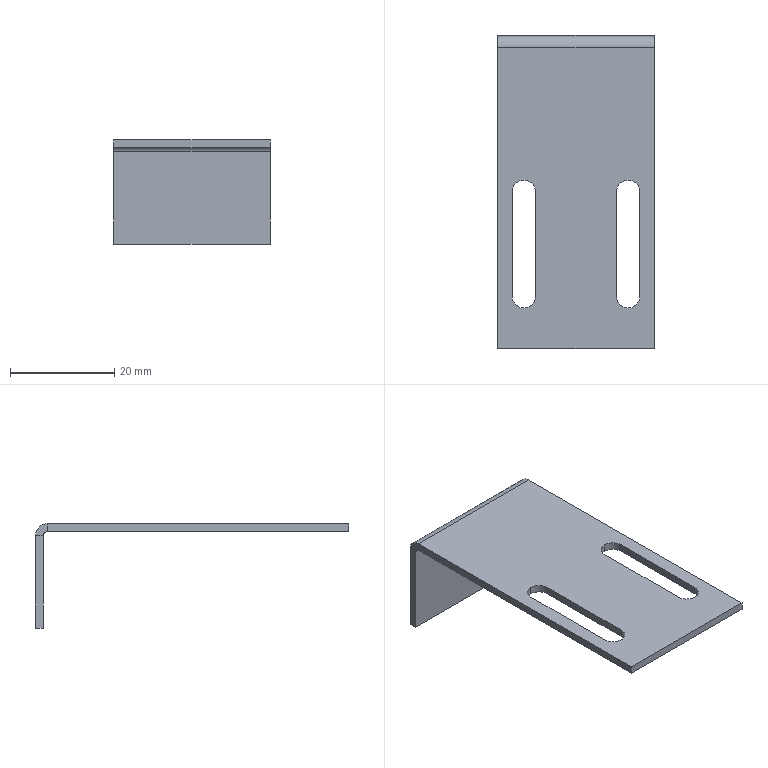Component | SolidWorks | SensorPlate-0510-1 | 1 solid | 24 faces | box 30 x 60 x 20 mm | volume 3186 mm3 | plane 16 | cylinder 8 | commonest cylinder face diameters 4.5 x6 4.473 x1 1.473 x1 | material 304
STEP:
#1=COLOUR_RGB('',0.7922,0.8196,0.9333);
#2=FILL_AREA_STYLE_COLOUR('',#1);
#3=FILL_AREA_STYLE('',(#2));
#4=SURFACE_STYLE_FILL_AREA(#3);
#5=SURFACE_SIDE_STYLE('',(#4));
#6=SURFACE_STYLE_USAGE(.BOTH.,#5);
#7=PRESENTATION_STYLE_ASSIGNMENT((#6));
#8=CARTESIAN_POINT('',(-85.441,9.356,136.319));
#9=VERTEX_POINT('',#8);
#10=CARTESIAN_POINT('',(-85.352,9.267,136.319));
#11=VERTEX_POINT('',#10);
#12=CARTESIAN_POINT('',(-85.441,9.267,136.319));
#13=DIRECTION('',(0.,0.,-1.));
#14=DIRECTION('',(0.,1.,0.));
#15=AXIS2_PLACEMENT_3D('',#12,#13,#14);
#16=CIRCLE('',#15,0.08858);
#17=EDGE_CURVE('',#9,#11,#16,.T.);
#18=ORIENTED_EDGE('',*,*,#17,.F.);
#19=CARTESIAN_POINT('',(-85.441,9.356,136.26));
#20=VERTEX_POINT('',#19);
#21=CARTESIAN_POINT('',(-85.441,9.356,136.319));
#22=DIRECTION('',(0.,0.,-1.));
#23=VECTOR('',#22,39.37);
#24=LINE('',#21,#23);
#25=EDGE_CURVE('',#9,#20,#24,.T.);
#26=ORIENTED_EDGE('',*,*,#25,.T.);
#27=CARTESIAN_POINT('',(-85.352,9.267,136.26));
#28=VERTEX_POINT('',#27);
#29=CARTESIAN_POINT('',(-85.441,9.267,136.26));
#30=DIRECTION('',(0.,0.,-1.));
#31=DIRECTION('',(0.,1.,0.));
#32=AXIS2_PLACEMENT_3D('',#29,#30,#31);
#33=CIRCLE('',#32,0.08858);
#34=EDGE_CURVE('',#20,#28,#33,.T.);
#35=ORIENTED_EDGE('',*,*,#34,.T.);
#36=CARTESIAN_POINT('',(-85.352,9.267,136.319));
#37=DIRECTION('',(0.,0.,-1.));
#38=VECTOR('',#37,39.37);
#39=LINE('',#36,#38);
#40=EDGE_CURVE('',#11,#28,#39,.T.);
#41=ORIENTED_EDGE('',*,*,#40,.F.);
#42=EDGE_LOOP('',(#18,#26,#35,#41));
#43=FACE_OUTER_BOUND('',#42,.T.);
#44=CARTESIAN_POINT('',(-85.441,9.267,136.319));
#45=DIRECTION('',(0.,0.,-1.));
#46=DIRECTION('',(0.,1.,0.));
#47=AXIS2_PLACEMENT_3D('',#44,#45,#46);
#48=CYLINDRICAL_SURFACE('',#47,0.08858);
#49=ADVANCED_FACE('',(#43),#48,.F.);
#50=CARTESIAN_POINT('',(-84.654,9.356,136.319));
#51=VERTEX_POINT('',#50);
#52=CARTESIAN_POINT('',(-84.565,9.267,136.319));
#53=VERTEX_POINT('',#52);
#54=CARTESIAN_POINT('',(-84.654,9.267,136.319));
#55=DIRECTION('',(0.,0.,-1.));
#56=DIRECTION('',(0.,-1.,0.));
#57=AXIS2_PLACEMENT_3D('',#54,#55,#56);
#58=CIRCLE('',#57,0.08858);
#59=EDGE_CURVE('',#51,#53,#58,.T.);
#60=ORIENTED_EDGE('',*,*,#59,.F.);
#61=CARTESIAN_POINT('',(-84.654,9.356,136.26));
#62=VERTEX_POINT('',#61);
#63=CARTESIAN_POINT('',(-84.654,9.356,136.319));
#64=DIRECTION('',(0.,0.,-1.));
#65=VECTOR('',#64,39.37);
#66=LINE('',#63,#65);
#67=EDGE_CURVE('',#51,#62,#66,.T.);
#68=ORIENTED_EDGE('',*,*,#67,.T.);
#69=CARTESIAN_POINT('',(-84.565,9.267,136.26));
#70=VERTEX_POINT('',#69);
#71=CARTESIAN_POINT('',(-84.654,9.267,136.26));
#72=DIRECTION('',(0.,0.,-1.));
#73=DIRECTION('',(0.,-1.,0.));
#74=AXIS2_PLACEMENT_3D('',#71,#72,#73);
#75=CIRCLE('',#74,0.08858);
#76=EDGE_CURVE('',#62,#70,#75,.T.);
#77=ORIENTED_EDGE('',*,*,#76,.T.);
#78=CARTESIAN_POINT('',(-84.565,9.267,136.319));
#79=DIRECTION('',(0.,0.,-1.));
#80=VECTOR('',#79,39.37);
#81=LINE('',#78,#80);
#82=EDGE_CURVE('',#53,#70,#81,.T.);
#83=ORIENTED_EDGE('',*,*,#82,.F.);
#84=EDGE_LOOP('',(#60,#68,#77,#83));
#85=FACE_OUTER_BOUND('',#84,.T.);
#86=CARTESIAN_POINT('',(-84.654,9.267,136.319));
#87=DIRECTION('',(0.,0.,-1.));
#88=DIRECTION('',(0.,1.,0.));
#89=AXIS2_PLACEMENT_3D('',#86,#87,#88);
#90=CYLINDRICAL_SURFACE('',#89,0.08858);
#91=ADVANCED_FACE('',(#85),#90,.F.);
#92=CARTESIAN_POINT('',(-85.638,10.36,136.319));
#93=VERTEX_POINT('',#92);
#94=CARTESIAN_POINT('',(-85.638,10.36,136.26));
#95=VERTEX_POINT('',#94);
#96=CARTESIAN_POINT('',(-85.638,10.36,136.319));
#97=DIRECTION('',(0.,0.,-1.));
#98=VECTOR('',#97,39.37);
#99=LINE('',#96,#98);
#100=EDGE_CURVE('',#93,#95,#99,.T.);
#101=ORIENTED_EDGE('',*,*,#100,.F.);
#102=CARTESIAN_POINT('',(-85.638,10.448,136.231));
#103=VERTEX_POINT('',#102);
#104=CARTESIAN_POINT('',(-85.638,10.36,136.231));
#105=DIRECTION('',(1.,-0.,0.));
#106=DIRECTION('',(0.,-1.,0.));
#107=AXIS2_PLACEMENT_3D('',#104,#105,#106);
#108=CIRCLE('',#107,0.08806);
#109=EDGE_CURVE('',#103,#93,#108,.T.);
#110=ORIENTED_EDGE('',*,*,#109,.F.);
#111=CARTESIAN_POINT('',(-85.638,10.389,136.231));
#112=VERTEX_POINT('',#111);
#113=CARTESIAN_POINT('',(-85.638,10.389,136.231));
#114=DIRECTION('',(0.,1.,0.));
#115=VECTOR('',#114,39.37);
#116=LINE('',#113,#115);
#117=EDGE_CURVE('',#112,#103,#116,.T.);
#118=ORIENTED_EDGE('',*,*,#117,.F.);
#119=CARTESIAN_POINT('',(-85.638,10.36,136.231));
#120=DIRECTION('',(1.,-0.,0.));
#121=DIRECTION('',(0.,0.,1.));
#122=AXIS2_PLACEMENT_3D('',#119,#120,#121);
#123=CIRCLE('',#122,0.029);
#124=EDGE_CURVE('',#112,#95,#123,.T.);
#125=ORIENTED_EDGE('',*,*,#124,.T.);
#126=EDGE_LOOP('',(#101,#110,#118,#125));
#127=FACE_OUTER_BOUND('',#126,.T.);
#128=CARTESIAN_POINT('',(-85.638,10.36,136.319));
#129=DIRECTION('',(-1.,0.,0.));
#130=DIRECTION('',(-0.,-1.,0.));
#131=AXIS2_PLACEMENT_3D('',#128,#129,#130);
#132=PLANE('',#131);
#133=ADVANCED_FACE('',(#127),#132,.T.);
#134=CARTESIAN_POINT('',(-85.638,8.086,136.319));
#135=VERTEX_POINT('',#134);
#136=CARTESIAN_POINT('',(-85.638,10.448,136.319));
#137=DIRECTION('',(-0.,-1.,0.));
#138=VECTOR('',#137,39.37);
#139=LINE('',#136,#138);
#140=EDGE_CURVE('',#93,#135,#139,.T.);
#141=ORIENTED_EDGE('',*,*,#140,.F.);
#142=ORIENTED_EDGE('',*,*,#100,.T.);
#143=CARTESIAN_POINT('',(-85.638,8.086,136.26));
#144=VERTEX_POINT('',#143);
#145=CARTESIAN_POINT('',(-85.638,10.448,136.26));
#146=DIRECTION('',(-0.,-1.,0.));
#147=VECTOR('',#146,39.37);
#148=LINE('',#145,#147);
#149=EDGE_CURVE('',#95,#144,#148,.T.);
#150=ORIENTED_EDGE('',*,*,#149,.T.);
#151=CARTESIAN_POINT('',(-85.638,8.086,136.26));
#152=DIRECTION('',(0.,0.,1.));
#153=VECTOR('',#152,39.37);
#154=LINE('',#151,#153);
#155=EDGE_CURVE('',#144,#135,#154,.T.);
#156=ORIENTED_EDGE('',*,*,#155,.T.);
#157=EDGE_LOOP('',(#141,#142,#150,#156));
#158=FACE_OUTER_BOUND('',#157,.T.);
#159=CARTESIAN_POINT('',(-85.638,10.389,136.231));
#160=DIRECTION('',(-1.,0.,0.));
#161=DIRECTION('',(-0.,-1.,0.));
#162=AXIS2_PLACEMENT_3D('',#159,#160,#161);
#163=PLANE('',#162);
#164=ADVANCED_FACE('',(#158),#163,.T.);
#165=CARTESIAN_POINT('',(-84.457,10.448,136.231));
#166=VERTEX_POINT('',#165);
#167=CARTESIAN_POINT('',(-84.457,10.389,136.231));
#168=VERTEX_POINT('',#167);
#169=CARTESIAN_POINT('',(-84.457,10.448,136.231));
#170=DIRECTION('',(-0.,-1.,0.));
#171=VECTOR('',#170,39.37);
#172=LINE('',#169,#171);
#173=EDGE_CURVE('',#166,#168,#172,.T.);
#174=ORIENTED_EDGE('',*,*,#173,.F.);
#175=CARTESIAN_POINT('',(-84.457,10.36,136.319));
#176=VERTEX_POINT('',#175);
#177=CARTESIAN_POINT('',(-84.457,10.36,136.231));
#178=DIRECTION('',(1.,-0.,0.));
#179=DIRECTION('',(0.,-1.,0.));
#180=AXIS2_PLACEMENT_3D('',#177,#178,#179);
#181=CIRCLE('',#180,0.08806);
#182=EDGE_CURVE('',#166,#176,#181,.T.);
#183=ORIENTED_EDGE('',*,*,#182,.T.);
#184=CARTESIAN_POINT('',(-84.457,10.36,136.26));
#185=VERTEX_POINT('',#184);
#186=CARTESIAN_POINT('',(-84.457,10.36,136.26));
#187=DIRECTION('',(0.,0.,1.));
#188=VECTOR('',#187,39.37);
#189=LINE('',#186,#188);
#190=EDGE_CURVE('',#185,#176,#189,.T.);
#191=ORIENTED_EDGE('',*,*,#190,.F.);
#192=CARTESIAN_POINT('',(-84.457,10.36,136.231));
#193=DIRECTION('',(1.,-0.,0.));
#194=DIRECTION('',(0.,0.,1.));
#195=AXIS2_PLACEMENT_3D('',#192,#193,#194);
#196=CIRCLE('',#195,0.029);
#197=EDGE_CURVE('',#168,#185,#196,.T.);
#198=ORIENTED_EDGE('',*,*,#197,.F.);
#199=EDGE_LOOP('',(#174,#183,#191,#198));
#200=FACE_OUTER_BOUND('',#199,.T.);
#201=CARTESIAN_POINT('',(-84.457,10.448,136.231));
#202=DIRECTION('',(1.,-0.,0.));
#203=DIRECTION('',(0.,1.,0.));
#204=AXIS2_PLACEMENT_3D('',#201,#202,#203);
#205=PLANE('',#204);
#206=ADVANCED_FACE('',(#200),#205,.T.);
#207=CARTESIAN_POINT('',(-84.457,10.448,135.531));
#208=VERTEX_POINT('',#207);
#209=CARTESIAN_POINT('',(-84.457,10.448,135.531));
#210=DIRECTION('',(0.,0.,1.));
#211=VECTOR('',#210,39.37);
#212=LINE('',#209,#211);
#213=EDGE_CURVE('',#208,#166,#212,.T.);
#214=ORIENTED_EDGE('',*,*,#213,.T.);
#215=ORIENTED_EDGE('',*,*,#173,.T.);
#216=CARTESIAN_POINT('',(-84.457,10.389,135.531));
#217=VERTEX_POINT('',#216);
#218=CARTESIAN_POINT('',(-84.457,10.389,135.531));
#219=DIRECTION('',(0.,0.,1.));
#220=VECTOR('',#219,39.37);
#221=LINE('',#218,#220);
#222=EDGE_CURVE('',#217,#168,#221,.T.);
#223=ORIENTED_EDGE('',*,*,#222,.F.);
#224=CARTESIAN_POINT('',(-84.457,10.448,135.531));
#225=DIRECTION('',(-0.,-1.,0.));
#226=VECTOR('',#225,39.37);
#227=LINE('',#224,#226);
#228=EDGE_CURVE('',#208,#217,#227,.T.);
#229=ORIENTED_EDGE('',*,*,#228,.F.);
#230=EDGE_LOOP('',(#214,#215,#223,#229));
#231=FACE_OUTER_BOUND('',#230,.T.);
#232=CARTESIAN_POINT('',(-84.457,10.36,136.26));
#233=DIRECTION('',(1.,-0.,0.));
#234=DIRECTION('',(0.,1.,0.));
#235=AXIS2_PLACEMENT_3D('',#232,#233,#234);
#236=PLANE('',#235);
#237=ADVANCED_FACE('',(#231),#236,.T.);
#238=CARTESIAN_POINT('',(-85.53,9.267,136.319));
#239=VERTEX_POINT('',#238);
#240=CARTESIAN_POINT('',(-85.441,9.267,136.319));
#241=DIRECTION('',(0.,0.,-1.));
#242=DIRECTION('',(0.,1.,0.));
#243=AXIS2_PLACEMENT_3D('',#240,#241,#242);
#244=CIRCLE('',#243,0.08858);
#245=EDGE_CURVE('',#239,#9,#244,.T.);
#246=ORIENTED_EDGE('',*,*,#245,.T.);
#247=ORIENTED_EDGE('',*,*,#17,.T.);
#248=CARTESIAN_POINT('',(-85.352,8.48,136.319));
#249=VERTEX_POINT('',#248);
#250=CARTESIAN_POINT('',(-85.352,9.267,136.319));
#251=DIRECTION('',(-0.,-1.,0.));
#252=VECTOR('',#251,39.37);
#253=LINE('',#250,#252);
#254=EDGE_CURVE('',#11,#249,#253,.T.);
#255=ORIENTED_EDGE('',*,*,#254,.T.);
#256=CARTESIAN_POINT('',(-85.53,8.48,136.319));
#257=VERTEX_POINT('',#256);
#258=CARTESIAN_POINT('',(-85.441,8.48,136.319));
#259=DIRECTION('',(0.,0.,-1.));
#260=DIRECTION('',(0.,1.,0.));
#261=AXIS2_PLACEMENT_3D('',#258,#259,#260);
#262=CIRCLE('',#261,0.08858);
#263=EDGE_CURVE('',#249,#257,#262,.T.);
#264=ORIENTED_EDGE('',*,*,#263,.T.);
#265=CARTESIAN_POINT('',(-85.53,9.267,136.319));
#266=DIRECTION('',(0.,1.,0.));
#267=VECTOR('',#266,39.37);
#268=LINE('',#265,#267);
#269=EDGE_CURVE('',#257,#239,#268,.T.);
#270=ORIENTED_EDGE('',*,*,#269,.T.);
#271=EDGE_LOOP('',(#246,#247,#255,#264,#270));
#272=FACE_BOUND('',#271,.T.);
#273=CARTESIAN_POINT('',(-84.742,9.267,136.319));
#274=VERTEX_POINT('',#273);
#275=CARTESIAN_POINT('',(-84.654,9.267,136.319));
#276=DIRECTION('',(0.,0.,-1.));
#277=DIRECTION('',(0.,-1.,0.));
#278=AXIS2_PLACEMENT_3D('',#275,#276,#277);
#279=CIRCLE('',#278,0.08858);
#280=EDGE_CURVE('',#274,#51,#279,.T.);
#281=ORIENTED_EDGE('',*,*,#280,.T.);
#282=ORIENTED_EDGE('',*,*,#59,.T.);
#283=CARTESIAN_POINT('',(-84.565,8.48,136.319));
#284=VERTEX_POINT('',#283);
#285=CARTESIAN_POINT('',(-84.565,9.267,136.319));
#286=DIRECTION('',(-0.,-1.,0.));
#287=VECTOR('',#286,39.37);
#288=LINE('',#285,#287);
#289=EDGE_CURVE('',#53,#284,#288,.T.);
#290=ORIENTED_EDGE('',*,*,#289,.T.);
#291=CARTESIAN_POINT('',(-84.742,8.48,136.319));
#292=VERTEX_POINT('',#291);
#293=CARTESIAN_POINT('',(-84.654,8.48,136.319));
#294=DIRECTION('',(0.,0.,-1.));
#295=DIRECTION('',(0.,-1.,0.));
#296=AXIS2_PLACEMENT_3D('',#293,#294,#295);
#297=CIRCLE('',#296,0.08858);
#298=EDGE_CURVE('',#284,#292,#297,.T.);
#299=ORIENTED_EDGE('',*,*,#298,.T.);
#300=CARTESIAN_POINT('',(-84.742,9.267,136.319));
#301=DIRECTION('',(0.,1.,0.));
#302=VECTOR('',#301,39.37);
#303=LINE('',#300,#302);
#304=EDGE_CURVE('',#292,#274,#303,.T.);
#305=ORIENTED_EDGE('',*,*,#304,.T.);
#306=EDGE_LOOP('',(#281,#282,#290,#299,#305));
#307=FACE_BOUND('',#306,.T.);
#308=CARTESIAN_POINT('',(-84.457,8.086,136.319));
#309=VERTEX_POINT('',#308);
#310=CARTESIAN_POINT('',(-84.457,10.448,136.319));
#311=DIRECTION('',(-0.,-1.,0.));
#312=VECTOR('',#311,39.37);
#313=LINE('',#310,#312);
#314=EDGE_CURVE('',#176,#309,#313,.T.);
#315=ORIENTED_EDGE('',*,*,#314,.F.);
#316=CARTESIAN_POINT('',(-85.638,10.36,136.319));
#317=DIRECTION('',(1.,-0.,0.));
#318=VECTOR('',#317,39.37);
#319=LINE('',#316,#318);
#320=EDGE_CURVE('',#93,#176,#319,.T.);
#321=ORIENTED_EDGE('',*,*,#320,.F.);
#322=ORIENTED_EDGE('',*,*,#140,.T.);
#323=CARTESIAN_POINT('',(-85.638,8.086,136.319));
#324=DIRECTION('',(1.,-0.,0.));
#325=VECTOR('',#324,39.37);
#326=LINE('',#323,#325);
#327=EDGE_CURVE('',#135,#309,#326,.T.);
#328=ORIENTED_EDGE('',*,*,#327,.T.);
#329=EDGE_LOOP('',(#315,#321,#322,#328));
#330=FACE_OUTER_BOUND('',#329,.T.);
#331=CARTESIAN_POINT('',(-85.638,10.448,136.319));
#332=DIRECTION('',(0.,0.,1.));
#333=DIRECTION('',(-0.,-1.,0.));
#334=AXIS2_PLACEMENT_3D('',#331,#332,#333);
#335=PLANE('',#334);
#336=ADVANCED_FACE('',(#272,#307,#330),#335,.T.);
#337=ORIENTED_EDGE('',*,*,#182,.F.);
#338=CARTESIAN_POINT('',(-85.638,10.448,136.231));
#339=DIRECTION('',(1.,-0.,0.));
#340=VECTOR('',#339,39.37);
#341=LINE('',#338,#340);
#342=EDGE_CURVE('',#103,#166,#341,.T.);
#343=ORIENTED_EDGE('',*,*,#342,.F.);
#344=ORIENTED_EDGE('',*,*,#109,.T.);
#345=ORIENTED_EDGE('',*,*,#320,.T.);
#346=EDGE_LOOP('',(#337,#343,#344,#345));
#347=FACE_OUTER_BOUND('',#346,.T.);
#348=CARTESIAN_POINT('',(-85.638,10.36,136.231));
#349=DIRECTION('',(1.,-0.,0.));
#350=DIRECTION('',(0.,1.,0.));
#351=AXIS2_PLACEMENT_3D('',#348,#349,#350);
#352=CYLINDRICAL_SURFACE('',#351,0.08806);
#353=ADVANCED_FACE('',(#347),#352,.T.);
#354=ORIENTED_EDGE('',*,*,#213,.F.);
#355=CARTESIAN_POINT('',(-85.638,10.448,135.531));
#356=VERTEX_POINT('',#355);
#357=CARTESIAN_POINT('',(-85.638,10.448,135.531));
#358=DIRECTION('',(1.,-0.,0.));
#359=VECTOR('',#358,39.37);
#360=LINE('',#357,#359);
#361=EDGE_CURVE('',#356,#208,#360,.T.);
#362=ORIENTED_EDGE('',*,*,#361,.F.);
#363=CARTESIAN_POINT('',(-85.638,10.448,135.531));
#364=DIRECTION('',(0.,0.,1.));
#365=VECTOR('',#364,39.37);
#366=LINE('',#363,#365);
#367=EDGE_CURVE('',#356,#103,#366,.T.);
#368=ORIENTED_EDGE('',*,*,#367,.T.);
#369=ORIENTED_EDGE('',*,*,#342,.T.);
#370=EDGE_LOOP('',(#354,#362,#368,#369));
#371=FACE_OUTER_BOUND('',#370,.T.);
#372=CARTESIAN_POINT('',(-85.638,10.448,135.531));
#373=DIRECTION('',(0.,1.,0.));
#374=DIRECTION('',(0.,0.,1.));
#375=AXIS2_PLACEMENT_3D('',#372,#373,#374);
#376=PLANE('',#375);
#377=ADVANCED_FACE('',(#371),#376,.T.);
#378=ORIENTED_EDGE('',*,*,#228,.T.);
#379=CARTESIAN_POINT('',(-85.638,10.389,135.531));
#380=VERTEX_POINT('',#379);
#381=CARTESIAN_POINT('',(-85.638,10.389,135.531));
#382=DIRECTION('',(1.,-0.,0.));
#383=VECTOR('',#382,39.37);
#384=LINE('',#381,#383);
#385=EDGE_CURVE('',#380,#217,#384,.T.);
#386=ORIENTED_EDGE('',*,*,#385,.F.);
#387=CARTESIAN_POINT('',(-85.638,10.448,135.531));
#388=DIRECTION('',(-0.,-1.,0.));
#389=VECTOR('',#388,39.37);
#390=LINE('',#387,#389);
#391=EDGE_CURVE('',#356,#380,#390,.T.);
#392=ORIENTED_EDGE('',*,*,#391,.F.);
#393=ORIENTED_EDGE('',*,*,#361,.T.);
#394=EDGE_LOOP('',(#378,#386,#392,#393));
#395=FACE_OUTER_BOUND('',#394,.T.);
#396=CARTESIAN_POINT('',(-85.638,10.448,135.531));
#397=DIRECTION('',(0.,0.,1.));
#398=DIRECTION('',(-0.,-1.,0.));
#399=AXIS2_PLACEMENT_3D('',#396,#397,#398);
#400=PLANE('',#399);
#401=ADVANCED_FACE('',(#395),#400,.F.);
#402=ORIENTED_EDGE('',*,*,#222,.T.);
#403=CARTESIAN_POINT('',(-85.638,10.389,136.231));
#404=DIRECTION('',(1.,-0.,0.));
#405=VECTOR('',#404,39.37);
#406=LINE('',#403,#405);
#407=EDGE_CURVE('',#112,#168,#406,.T.);
#408=ORIENTED_EDGE('',*,*,#407,.F.);
#409=CARTESIAN_POINT('',(-85.638,10.389,135.531));
#410=DIRECTION('',(0.,0.,1.));
#411=VECTOR('',#410,39.37);
#412=LINE('',#409,#411);
#413=EDGE_CURVE('',#380,#112,#412,.T.);
#414=ORIENTED_EDGE('',*,*,#413,.F.);
#415=ORIENTED_EDGE('',*,*,#385,.T.);
#416=EDGE_LOOP('',(#402,#408,#414,#415));
#417=FACE_OUTER_BOUND('',#416,.T.);
#418=CARTESIAN_POINT('',(-85.638,10.389,135.531));
#419=DIRECTION('',(0.,1.,0.));
#420=DIRECTION('',(0.,0.,1.));
#421=AXIS2_PLACEMENT_3D('',#418,#419,#420);
#422=PLANE('',#421);
#423=ADVANCED_FACE('',(#417),#422,.F.);
#424=ORIENTED_EDGE('',*,*,#197,.T.);
#425=CARTESIAN_POINT('',(-85.638,10.36,136.26));
#426=DIRECTION('',(1.,-0.,0.));
#427=VECTOR('',#426,39.37);
#428=LINE('',#425,#427);
#429=EDGE_CURVE('',#95,#185,#428,.T.);
#430=ORIENTED_EDGE('',*,*,#429,.F.);
#431=ORIENTED_EDGE('',*,*,#124,.F.);
#432=ORIENTED_EDGE('',*,*,#407,.T.);
#433=EDGE_LOOP('',(#424,#430,#431,#432));
#434=FACE_OUTER_BOUND('',#433,.T.);
#435=CARTESIAN_POINT('',(-85.638,10.36,136.231));
#436=DIRECTION('',(1.,-0.,0.));
#437=DIRECTION('',(0.,1.,0.));
#438=AXIS2_PLACEMENT_3D('',#435,#436,#437);
#439=CYLINDRICAL_SURFACE('',#438,0.029);
#440=ADVANCED_FACE('',(#434),#439,.F.);
#441=CARTESIAN_POINT('',(-85.352,8.48,136.26));
#442=VERTEX_POINT('',#441);
#443=CARTESIAN_POINT('',(-85.352,9.267,136.26));
#444=DIRECTION('',(-0.,-1.,0.));
#445=VECTOR('',#444,39.37);
#446=LINE('',#443,#445);
#447=EDGE_CURVE('',#28,#442,#446,.T.);
#448=ORIENTED_EDGE('',*,*,#447,.F.);
#449=ORIENTED_EDGE('',*,*,#34,.F.);
#450=CARTESIAN_POINT('',(-85.53,9.267,136.26));
#451=VERTEX_POINT('',#450);
#452=CARTESIAN_POINT('',(-85.441,9.267,136.26));
#453=DIRECTION('',(0.,0.,-1.));
#454=DIRECTION('',(0.,1.,0.));
#455=AXIS2_PLACEMENT_3D('',#452,#453,#454);
#456=CIRCLE('',#455,0.08858);
#457=EDGE_CURVE('',#451,#20,#456,.T.);
#458=ORIENTED_EDGE('',*,*,#457,.F.);
#459=CARTESIAN_POINT('',(-85.53,8.48,136.26));
#460=VERTEX_POINT('',#459);
#461=CARTESIAN_POINT('',(-85.53,9.267,136.26));
#462=DIRECTION('',(0.,1.,0.));
#463=VECTOR('',#462,39.37);
#464=LINE('',#461,#463);
#465=EDGE_CURVE('',#460,#451,#464,.T.);
#466=ORIENTED_EDGE('',*,*,#465,.F.);
#467=CARTESIAN_POINT('',(-85.441,8.48,136.26));
#468=DIRECTION('',(0.,0.,-1.));
#469=DIRECTION('',(0.,1.,0.));
#470=AXIS2_PLACEMENT_3D('',#467,#468,#469);
#471=CIRCLE('',#470,0.08858);
#472=EDGE_CURVE('',#442,#460,#471,.T.);
#473=ORIENTED_EDGE('',*,*,#472,.F.);
#474=EDGE_LOOP('',(#448,#449,#458,#466,#473));
#475=FACE_BOUND('',#474,.T.);
#476=CARTESIAN_POINT('',(-84.565,8.48,136.26));
#477=VERTEX_POINT('',#476);
#478=CARTESIAN_POINT('',(-84.565,9.267,136.26));
#479=DIRECTION('',(-0.,-1.,0.));
#480=VECTOR('',#479,39.37);
#481=LINE('',#478,#480);
#482=EDGE_CURVE('',#70,#477,#481,.T.);
#483=ORIENTED_EDGE('',*,*,#482,.F.);
#484=ORIENTED_EDGE('',*,*,#76,.F.);
#485=CARTESIAN_POINT('',(-84.742,9.267,136.26));
#486=VERTEX_POINT('',#485);
#487=CARTESIAN_POINT('',(-84.654,9.267,136.26));
#488=DIRECTION('',(0.,0.,-1.));
#489=DIRECTION('',(0.,-1.,0.));
#490=AXIS2_PLACEMENT_3D('',#487,#488,#489);
#491=CIRCLE('',#490,0.08858);
#492=EDGE_CURVE('',#486,#62,#491,.T.);
#493=ORIENTED_EDGE('',*,*,#492,.F.);
#494=CARTESIAN_POINT('',(-84.742,8.48,136.26));
#495=VERTEX_POINT('',#494);
#496=CARTESIAN_POINT('',(-84.742,9.267,136.26));
#497=DIRECTION('',(0.,1.,0.));
#498=VECTOR('',#497,39.37);
#499=LINE('',#496,#498);
#500=EDGE_CURVE('',#495,#486,#499,.T.);
#501=ORIENTED_EDGE('',*,*,#500,.F.);
#502=CARTESIAN_POINT('',(-84.654,8.48,136.26));
#503=DIRECTION('',(0.,0.,-1.));
#504=DIRECTION('',(0.,-1.,0.));
#505=AXIS2_PLACEMENT_3D('',#502,#503,#504);
#506=CIRCLE('',#505,0.08858);
#507=EDGE_CURVE('',#477,#495,#506,.T.);
#508=ORIENTED_EDGE('',*,*,#507,.F.);
#509=EDGE_LOOP('',(#483,#484,#493,#501,#508));
#510=FACE_BOUND('',#509,.T.);
#511=CARTESIAN_POINT('',(-84.457,8.086,136.26));
#512=VERTEX_POINT('',#511);
#513=CARTESIAN_POINT('',(-84.457,10.448,136.26));
#514=DIRECTION('',(-0.,-1.,0.));
#515=VECTOR('',#514,39.37);
#516=LINE('',#513,#515);
#517=EDGE_CURVE('',#185,#512,#516,.T.);
#518=ORIENTED_EDGE('',*,*,#517,.T.);
#519=CARTESIAN_POINT('',(-85.638,8.086,136.26));
#520=DIRECTION('',(1.,-0.,0.));
#521=VECTOR('',#520,39.37);
#522=LINE('',#519,#521);
#523=EDGE_CURVE('',#144,#512,#522,.T.);
#524=ORIENTED_EDGE('',*,*,#523,.F.);
#525=ORIENTED_EDGE('',*,*,#149,.F.);
#526=ORIENTED_EDGE('',*,*,#429,.T.);
#527=EDGE_LOOP('',(#518,#524,#525,#526));
#528=FACE_OUTER_BOUND('',#527,.T.);
#529=CARTESIAN_POINT('',(-85.638,10.448,136.26));
#530=DIRECTION('',(0.,0.,1.));
#531=DIRECTION('',(-0.,-1.,0.));
#532=AXIS2_PLACEMENT_3D('',#529,#530,#531);
#533=PLANE('',#532);
#534=ADVANCED_FACE('',(#475,#510,#528),#533,.F.);
#535=CARTESIAN_POINT('',(-84.457,8.086,136.26));
#536=DIRECTION('',(0.,0.,1.));
#537=VECTOR('',#536,39.37);
#538=LINE('',#535,#537);
#539=EDGE_CURVE('',#512,#309,#538,.T.);
#540=ORIENTED_EDGE('',*,*,#539,.T.);
#541=ORIENTED_EDGE('',*,*,#327,.F.);
#542=ORIENTED_EDGE('',*,*,#155,.F.);
#543=ORIENTED_EDGE('',*,*,#523,.T.);
#544=EDGE_LOOP('',(#540,#541,#542,#543));
#545=FACE_OUTER_BOUND('',#544,.T.);
#546=CARTESIAN_POINT('',(-85.638,8.086,136.26));
#547=DIRECTION('',(0.,1.,0.));
#548=DIRECTION('',(0.,0.,1.));
#549=AXIS2_PLACEMENT_3D('',#546,#547,#548);
#550=PLANE('',#549);
#551=ADVANCED_FACE('',(#545),#550,.F.);
#552=ORIENTED_EDGE('',*,*,#413,.T.);
#553=ORIENTED_EDGE('',*,*,#117,.T.);
#554=ORIENTED_EDGE('',*,*,#367,.F.);
#555=ORIENTED_EDGE('',*,*,#391,.T.);
#556=EDGE_LOOP('',(#552,#553,#554,#555));
#557=FACE_OUTER_BOUND('',#556,.T.);
#558=CARTESIAN_POINT('',(-85.638,10.36,136.231));
#559=DIRECTION('',(1.,-0.,0.));
#560=DIRECTION('',(0.,0.,1.));
#561=AXIS2_PLACEMENT_3D('',#558,#559,#560);
#562=PLANE('',#561);
#563=ADVANCED_FACE('',(#557),#562,.F.);
#564=ORIENTED_EDGE('',*,*,#314,.T.);
#565=ORIENTED_EDGE('',*,*,#539,.F.);
#566=ORIENTED_EDGE('',*,*,#517,.F.);
#567=ORIENTED_EDGE('',*,*,#190,.T.);
#568=EDGE_LOOP('',(#564,#565,#566,#567));
#569=FACE_OUTER_BOUND('',#568,.T.);
#570=CARTESIAN_POINT('',(-84.457,10.36,136.231));
#571=DIRECTION('',(1.,-0.,0.));
#572=DIRECTION('',(0.,0.,1.));
#573=AXIS2_PLACEMENT_3D('',#570,#571,#572);
#574=PLANE('',#573);
#575=ADVANCED_FACE('',(#569),#574,.T.);
#576=ORIENTED_EDGE('',*,*,#67,.F.);
#577=ORIENTED_EDGE('',*,*,#280,.F.);
#578=CARTESIAN_POINT('',(-84.742,9.267,136.319));
#579=DIRECTION('',(0.,0.,-1.));
#580=VECTOR('',#579,39.37);
#581=LINE('',#578,#580);
#582=EDGE_CURVE('',#274,#486,#581,.T.);
#583=ORIENTED_EDGE('',*,*,#582,.T.);
#584=ORIENTED_EDGE('',*,*,#492,.T.);
#585=EDGE_LOOP('',(#576,#577,#583,#584));
#586=FACE_OUTER_BOUND('',#585,.T.);
#587=CARTESIAN_POINT('',(-84.654,9.267,136.319));
#588=DIRECTION('',(0.,0.,-1.));
#589=DIRECTION('',(0.,1.,0.));
#590=AXIS2_PLACEMENT_3D('',#587,#588,#589);
#591=CYLINDRICAL_SURFACE('',#590,0.08858);
#592=ADVANCED_FACE('',(#586),#591,.F.);
#593=ORIENTED_EDGE('',*,*,#500,.T.);
#594=ORIENTED_EDGE('',*,*,#582,.F.);
#595=ORIENTED_EDGE('',*,*,#304,.F.);
#596=CARTESIAN_POINT('',(-84.742,8.48,136.319));
#597=DIRECTION('',(0.,0.,-1.));
#598=VECTOR('',#597,39.37);
#599=LINE('',#596,#598);
#600=EDGE_CURVE('',#292,#495,#599,.T.);
#601=ORIENTED_EDGE('',*,*,#600,.T.);
#602=EDGE_LOOP('',(#593,#594,#595,#601));
#603=FACE_OUTER_BOUND('',#602,.T.);
#604=CARTESIAN_POINT('',(-84.742,9.267,136.319));
#605=DIRECTION('',(-1.,0.,0.));
#606=DIRECTION('',(-0.,-1.,0.));
#607=AXIS2_PLACEMENT_3D('',#604,#605,#606);
#608=PLANE('',#607);
#609=ADVANCED_FACE('',(#603),#608,.F.);
#610=ORIENTED_EDGE('',*,*,#507,.T.);
#611=ORIENTED_EDGE('',*,*,#600,.F.);
#612=ORIENTED_EDGE('',*,*,#298,.F.);
#613=CARTESIAN_POINT('',(-84.565,8.48,136.319));
#614=DIRECTION('',(0.,0.,-1.));
#615=VECTOR('',#614,39.37);
#616=LINE('',#613,#615);
#617=EDGE_CURVE('',#284,#477,#616,.T.);
#618=ORIENTED_EDGE('',*,*,#617,.T.);
#619=EDGE_LOOP('',(#610,#611,#612,#618));
#620=FACE_OUTER_BOUND('',#619,.T.);
#621=CARTESIAN_POINT('',(-84.654,8.48,136.319));
#622=DIRECTION('',(0.,0.,-1.));
#623=DIRECTION('',(0.,1.,0.));
#624=AXIS2_PLACEMENT_3D('',#621,#622,#623);
#625=CYLINDRICAL_SURFACE('',#624,0.08858);
#626=ADVANCED_FACE('',(#620),#625,.F.);
#627=ORIENTED_EDGE('',*,*,#482,.T.);
#628=ORIENTED_EDGE('',*,*,#617,.F.);
#629=ORIENTED_EDGE('',*,*,#289,.F.);
#630=ORIENTED_EDGE('',*,*,#82,.T.);
#631=EDGE_LOOP('',(#627,#628,#629,#630));
#632=FACE_OUTER_BOUND('',#631,.T.);
#633=CARTESIAN_POINT('',(-84.565,9.267,136.319));
#634=DIRECTION('',(1.,-0.,0.));
#635=DIRECTION('',(0.,1.,0.));
#636=AXIS2_PLACEMENT_3D('',#633,#634,#635);
#637=PLANE('',#636);
#638=ADVANCED_FACE('',(#632),#637,.F.);
#639=ORIENTED_EDGE('',*,*,#25,.F.);
#640=ORIENTED_EDGE('',*,*,#245,.F.);
#641=CARTESIAN_POINT('',(-85.53,9.267,136.319));
#642=DIRECTION('',(0.,0.,-1.));
#643=VECTOR('',#642,39.37);
#644=LINE('',#641,#643);
#645=EDGE_CURVE('',#239,#451,#644,.T.);
#646=ORIENTED_EDGE('',*,*,#645,.T.);
#647=ORIENTED_EDGE('',*,*,#457,.T.);
#648=EDGE_LOOP('',(#639,#640,#646,#647));
#649=FACE_OUTER_BOUND('',#648,.T.);
#650=CARTESIAN_POINT('',(-85.441,9.267,136.319));
#651=DIRECTION('',(0.,0.,-1.));
#652=DIRECTION('',(0.,1.,0.));
#653=AXIS2_PLACEMENT_3D('',#650,#651,#652);
#654=CYLINDRICAL_SURFACE('',#653,0.08858);
#655=ADVANCED_FACE('',(#649),#654,.F.);
#656=ORIENTED_EDGE('',*,*,#465,.T.);
#657=ORIENTED_EDGE('',*,*,#645,.F.);
#658=ORIENTED_EDGE('',*,*,#269,.F.);
#659=CARTESIAN_POINT('',(-85.53,8.48,136.319));
#660=DIRECTION('',(0.,0.,-1.));
#661=VECTOR('',#660,39.37);
#662=LINE('',#659,#661);
#663=EDGE_CURVE('',#257,#460,#662,.T.);
#664=ORIENTED_EDGE('',*,*,#663,.T.);
#665=EDGE_LOOP('',(#656,#657,#658,#664));
#666=FACE_OUTER_BOUND('',#665,.T.);
#667=CARTESIAN_POINT('',(-85.53,9.267,136.319));
#668=DIRECTION('',(-1.,0.,0.));
#669=DIRECTION('',(-0.,-1.,0.));
#670=AXIS2_PLACEMENT_3D('',#667,#668,#669);
#671=PLANE('',#670);
#672=ADVANCED_FACE('',(#666),#671,.F.);
#673=ORIENTED_EDGE('',*,*,#472,.T.);
#674=ORIENTED_EDGE('',*,*,#663,.F.);
#675=ORIENTED_EDGE('',*,*,#263,.F.);
#676=CARTESIAN_POINT('',(-85.352,8.48,136.319));
#677=DIRECTION('',(0.,0.,-1.));
#678=VECTOR('',#677,39.37);
#679=LINE('',#676,#678);
#680=EDGE_CURVE('',#249,#442,#679,.T.);
#681=ORIENTED_EDGE('',*,*,#680,.T.);
#682=EDGE_LOOP('',(#673,#674,#675,#681));
#683=FACE_OUTER_BOUND('',#682,.T.);
#684=CARTESIAN_POINT('',(-85.441,8.48,136.319));
#685=DIRECTION('',(0.,0.,-1.));
#686=DIRECTION('',(0.,1.,0.));
#687=AXIS2_PLACEMENT_3D('',#684,#685,#686);
#688=CYLINDRICAL_SURFACE('',#687,0.08858);
#689=ADVANCED_FACE('',(#683),#688,.F.);
#690=ORIENTED_EDGE('',*,*,#447,.T.);
#691=ORIENTED_EDGE('',*,*,#680,.F.);
#692=ORIENTED_EDGE('',*,*,#254,.F.);
#693=ORIENTED_EDGE('',*,*,#40,.T.);
#694=EDGE_LOOP('',(#690,#691,#692,#693));
#695=FACE_OUTER_BOUND('',#694,.T.);
#696=CARTESIAN_POINT('',(-85.352,9.267,136.319));
#697=DIRECTION('',(1.,-0.,0.));
#698=DIRECTION('',(0.,1.,0.));
#699=AXIS2_PLACEMENT_3D('',#696,#697,#698);
#700=PLANE('',#699);
#701=ADVANCED_FACE('',(#695),#700,.F.);
#702=CLOSED_SHELL('',(#49,#91,#133,#164,#206,#237,#336,#353,#377,#401,#423,#440,#534,#551,#563,#575,#592,#609,#626,#638,#655,#672,#689,#701));
#703=MANIFOLD_SOLID_BREP('',#702);
#704=STYLED_ITEM('',(#7),#703);
#705=PRESENTATION_LAYER_ASSIGNMENT('','',(#704));
#706=CARTESIAN_POINT('',(0.,0.,0.));
#707=DIRECTION('',(0.,0.,1.));
#708=DIRECTION('',(1.,0.,0.));
#709=AXIS2_PLACEMENT_3D('',#706,#707,#708);
#710=(LENGTH_UNIT()NAMED_UNIT(*)SI_UNIT($,.METRE.));
#711=LENGTH_MEASURE_WITH_UNIT(LENGTH_MEASURE(0.0254),#710);
#712=DIMENSIONAL_EXPONENTS(1.,0.,0.,0.,0.,0.,0.);
#713=(CONVERSION_BASED_UNIT('',#711)LENGTH_UNIT()NAMED_UNIT(#712));
#714=UNCERTAINTY_MEASURE_WITH_UNIT(LENGTH_MEASURE(0.00001),#713,'','');
#715=(NAMED_UNIT(*)PLANE_ANGLE_UNIT()SI_UNIT($,.RADIAN.));
#716=(NAMED_UNIT(*)SI_UNIT($,.STERADIAN.)SOLID_ANGLE_UNIT());
#717=(GEOMETRIC_REPRESENTATION_CONTEXT(3)GLOBAL_UNCERTAINTY_ASSIGNED_CONTEXT((#714))GLOBAL_UNIT_ASSIGNED_CONTEXT((#713,#715,#716))REPRESENTATION_CONTEXT('',''));
#718=ADVANCED_BREP_SHAPE_REPRESENTATION('',(#703,#709),#717);
#719=(LENGTH_UNIT()NAMED_UNIT(*)SI_UNIT($,.METRE.));
#720=LENGTH_MEASURE_WITH_UNIT(LENGTH_MEASURE(0.0254),#719);
#721=DIMENSIONAL_EXPONENTS(1.,0.,0.,0.,0.,0.,0.);
#722=(CONVERSION_BASED_UNIT('',#720)LENGTH_UNIT()NAMED_UNIT(#721));
#723=UNCERTAINTY_MEASURE_WITH_UNIT(LENGTH_MEASURE(0.00001),#722,'','');
#724=(NAMED_UNIT(*)PLANE_ANGLE_UNIT()SI_UNIT($,.RADIAN.));
#725=(NAMED_UNIT(*)SI_UNIT($,.STERADIAN.)SOLID_ANGLE_UNIT());
#726=(GEOMETRIC_REPRESENTATION_CONTEXT(3)GLOBAL_UNCERTAINTY_ASSIGNED_CONTEXT((#723))GLOBAL_UNIT_ASSIGNED_CONTEXT((#722,#724,#725))REPRESENTATION_CONTEXT('',''));
#727=MECHANICAL_DESIGN_GEOMETRIC_PRESENTATION_REPRESENTATION('',(#704),#726);